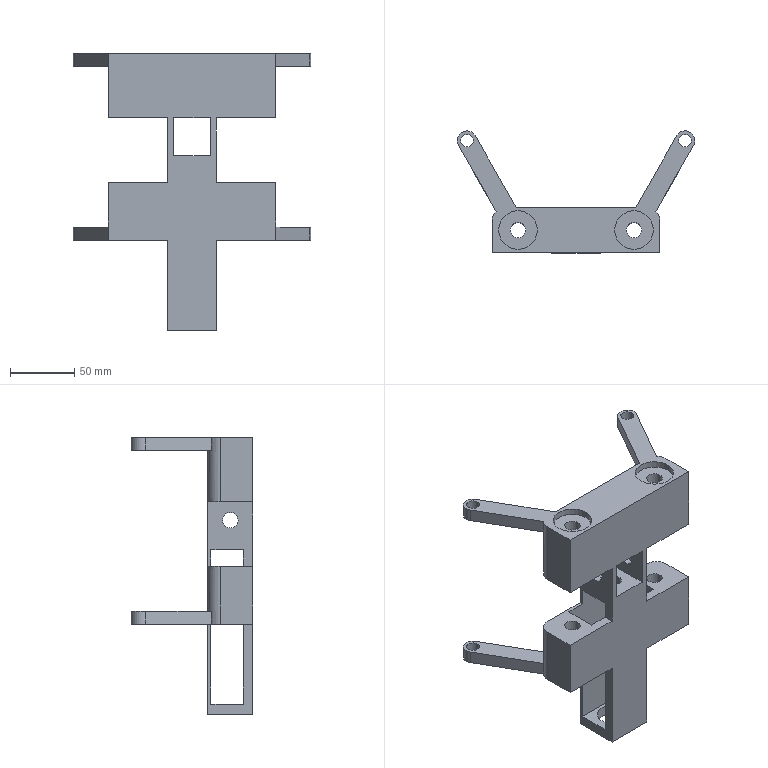Component | SolidWorks | MainBody-2 | 1 solid | 84 faces | volume 410843 mm3 | plane 44 | cylinder 40 | commonest cylinder face diameters 12 x14 10 x8 15 x6 20 x6 30 x4 25 x2